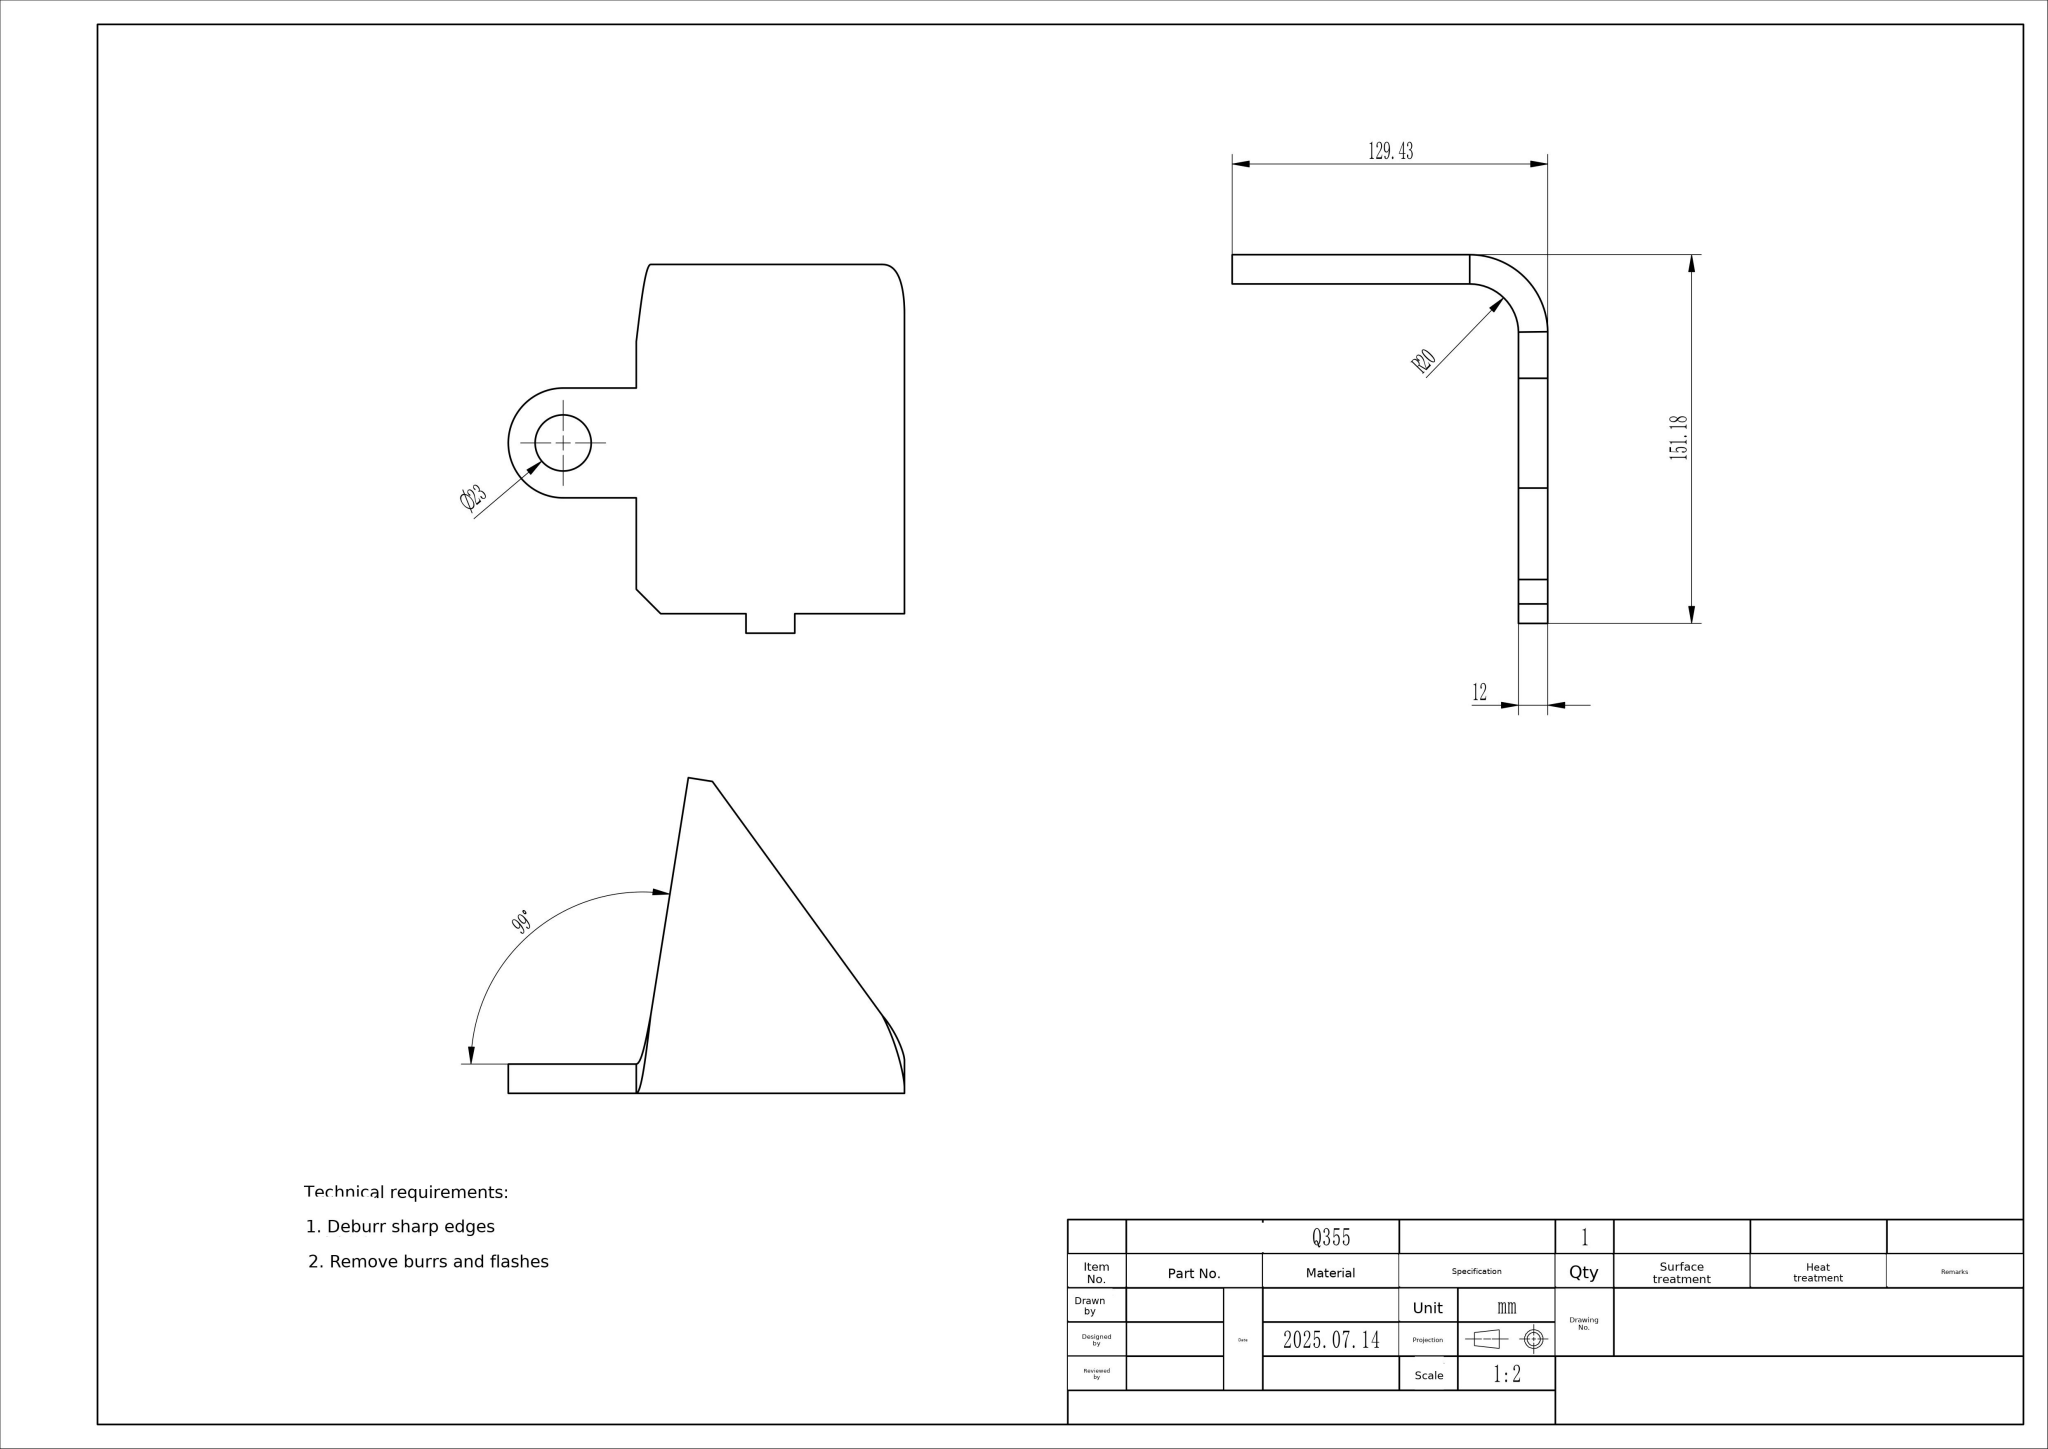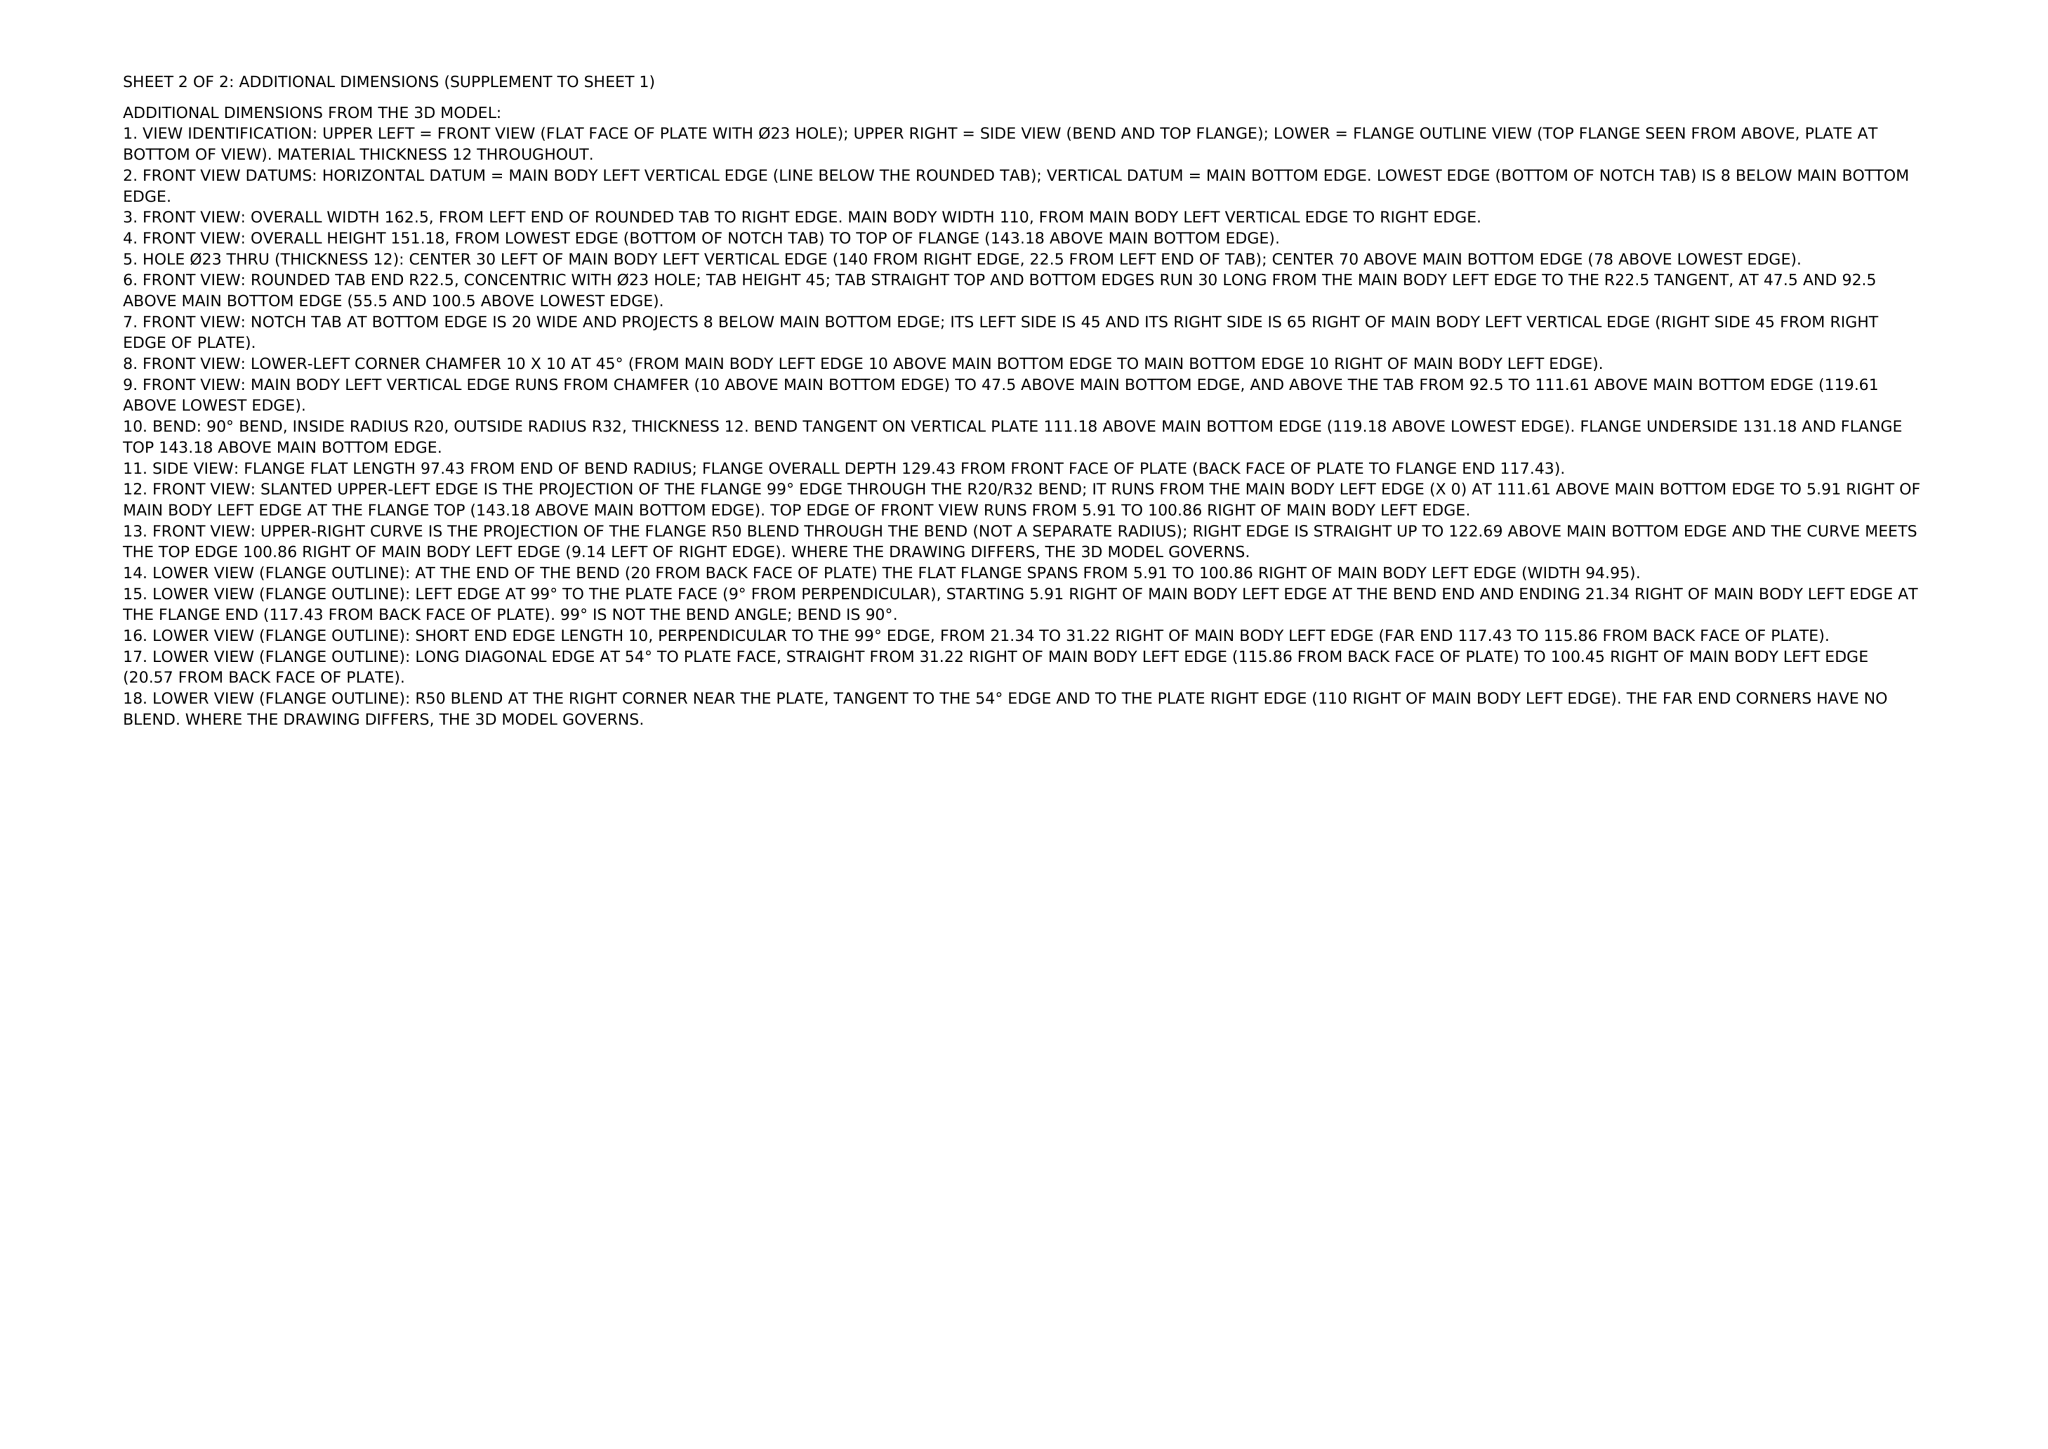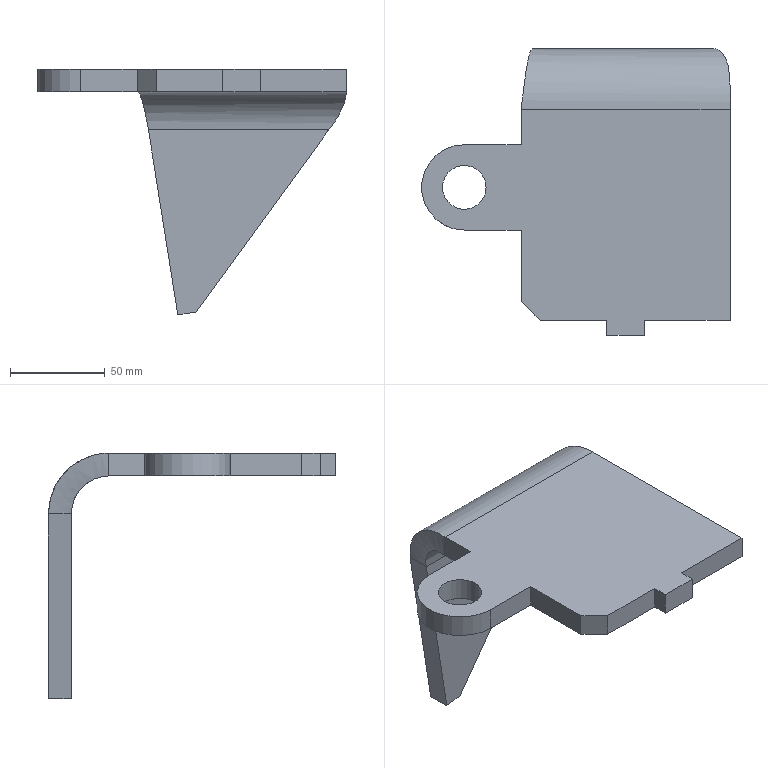Part | NX | mm | 1 solid | 25 faces | box 162.5 x 151.18 x 129.43 mm | volume 280745 mm3 | plane 18 | cylinder 5 | spline 2 | commonest cylinder face diameters 100 x1 23 x1 45 x1 64 x1 40 x1